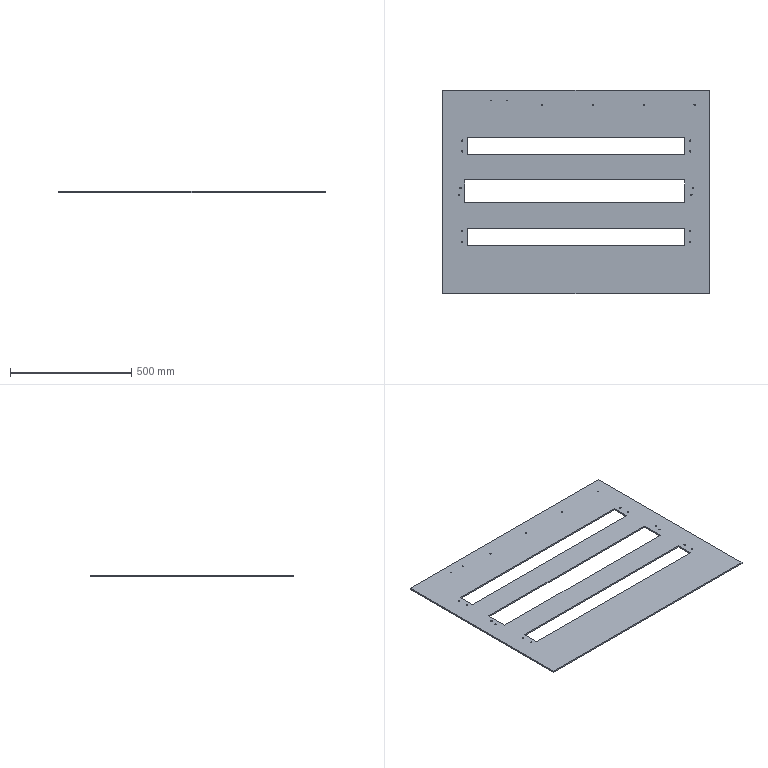Component | SolidWorks | DC-Motor-111-1 | 1 solid | 58 faces | box 1100 x 840 x 6 mm | volume 4253901 mm3 | cylinder 36 | plane 18 | cone 4 | commonest cylinder face diameters 5 x32 3.3 x4
build123d program:
from build123d import *

# Parameters (mm, degrees)
SKETCH1_W                   = 1100
SKETCH1_H                   = 840
BOSS_EXTRUDE1_DEPTH         = 3
SKETCH2_W                   = 910
SKETCH2_H                   = 93.5
CUT_EXTRUDE1_DEPTH          = 540
SKETCH3_W                   = 900
SKETCH3_H                   = 72
CUT_EXTRUDE2_DEPTH          = 695
M6_TAPPED_HOLE1_D           = 5
M6_TAPPED_HOLE2_D           = 5
M4_TAPPED_HOLE1_D           = 3.3
M4_TAPPED_HOLE1_CSINK_D     = 4.05
M4_TAPPED_HOLE1_CSINK_ANGLE = 90
M6_TAPPED_HOLE3_D           = 5


with BuildPart() as part:
    # Sketch1 → Boss-Extrude1 (new, symmetric)
    with BuildSketch(Plane.XY):
        Rectangle(SKETCH1_W, SKETCH1_H)
    extrude(amount=BOSS_EXTRUDE1_DEPTH, both=True)

    # Sketch2 → Cut-Extrude1 (cut)
    with BuildSketch(Plane(origin=(0, 0, -69), x_dir=(-1, 0, 0), z_dir=(0, 0, -1))):
        with Locations((5, 3.25)):
            Rectangle(SKETCH2_W, SKETCH2_H)
    extrude(amount=-CUT_EXTRUDE1_DEPTH, mode=Mode.SUBTRACT)

    # Sketch3 → Cut-Extrude2 (cut)
    with BuildSketch(Plane.XY.offset(3)):
        with Locations((0, -185)):
            Rectangle(SKETCH3_W, SKETCH3_H)
        with Locations((0, 190)):
            Rectangle(SKETCH3_W, SKETCH3_H)
    extrude(amount=-CUT_EXTRUDE2_DEPTH, mode=Mode.SUBTRACT)

    # M6 Tapped Hole1 (through all)
    with Locations(Plane.XY.offset(3)):
        with Locations((-477, 16.5), (-482, -11.5), (482, 16.5), (477, -11.5)):
            Hole(M6_TAPPED_HOLE1_D / 2)

    # M6 Tapped Hole2 (through all)
    with Locations(Plane.XY.offset(3)):
        with Locations((-470, 212.5), (-470, 167.5), (-470, -162.5), (-470, -207.5), (472, 212.5), (472, 167.5), (472, -162.5), (472, -207.5)):
            Hole(M6_TAPPED_HOLE2_D / 2)

    # M4 Tapped Hole1 (through all)
    with Locations(Plane(origin=(0, 0, -3), x_dir=(-1, 0, 0), z_dir=(0, 0, -1))):
        with Locations((351, 378), (284, 378)):
            CounterSinkHole(M4_TAPPED_HOLE1_D / 2, M4_TAPPED_HOLE1_CSINK_D / 2, counter_sink_angle=M4_TAPPED_HOLE1_CSINK_ANGLE)

    # M6 Tapped Hole3 (through all)
    with Locations(Plane(origin=(0, 0, -3), x_dir=(-1, 0, 0), z_dir=(0, 0, -1))):
        with Locations((-490, 360), (-280, 360), (-70, 360), (140, 360)):
            Hole(M6_TAPPED_HOLE3_D / 2)


solid = part.part

# Placed as in the assembly
solid = solid.moved(Location((2.208, 11.801, -423), (0, 0, 0)))